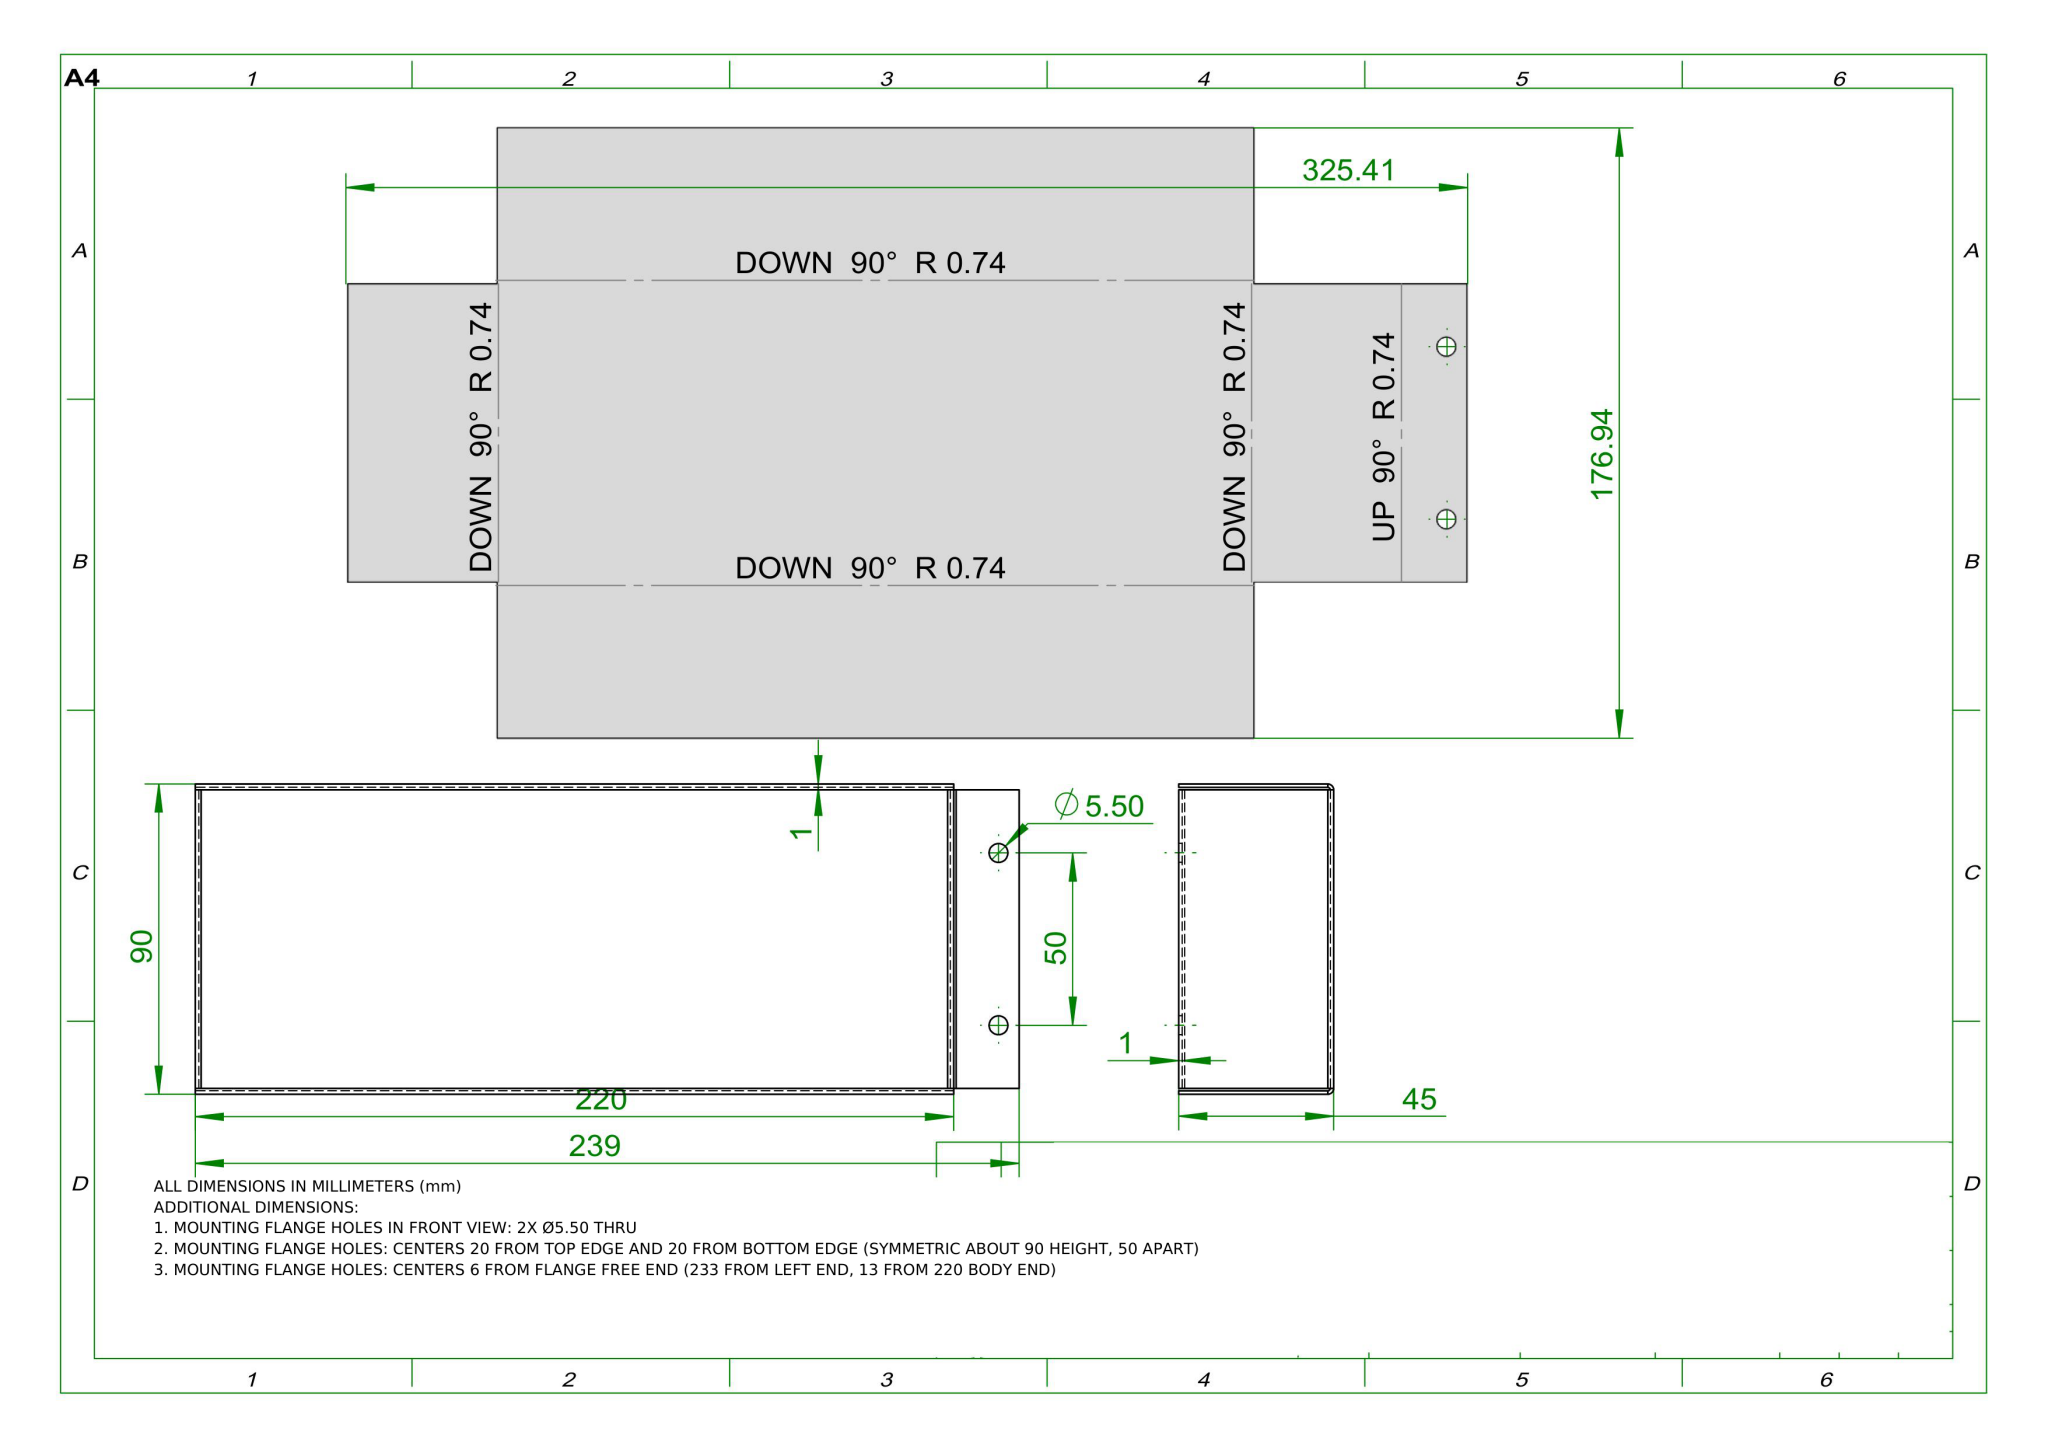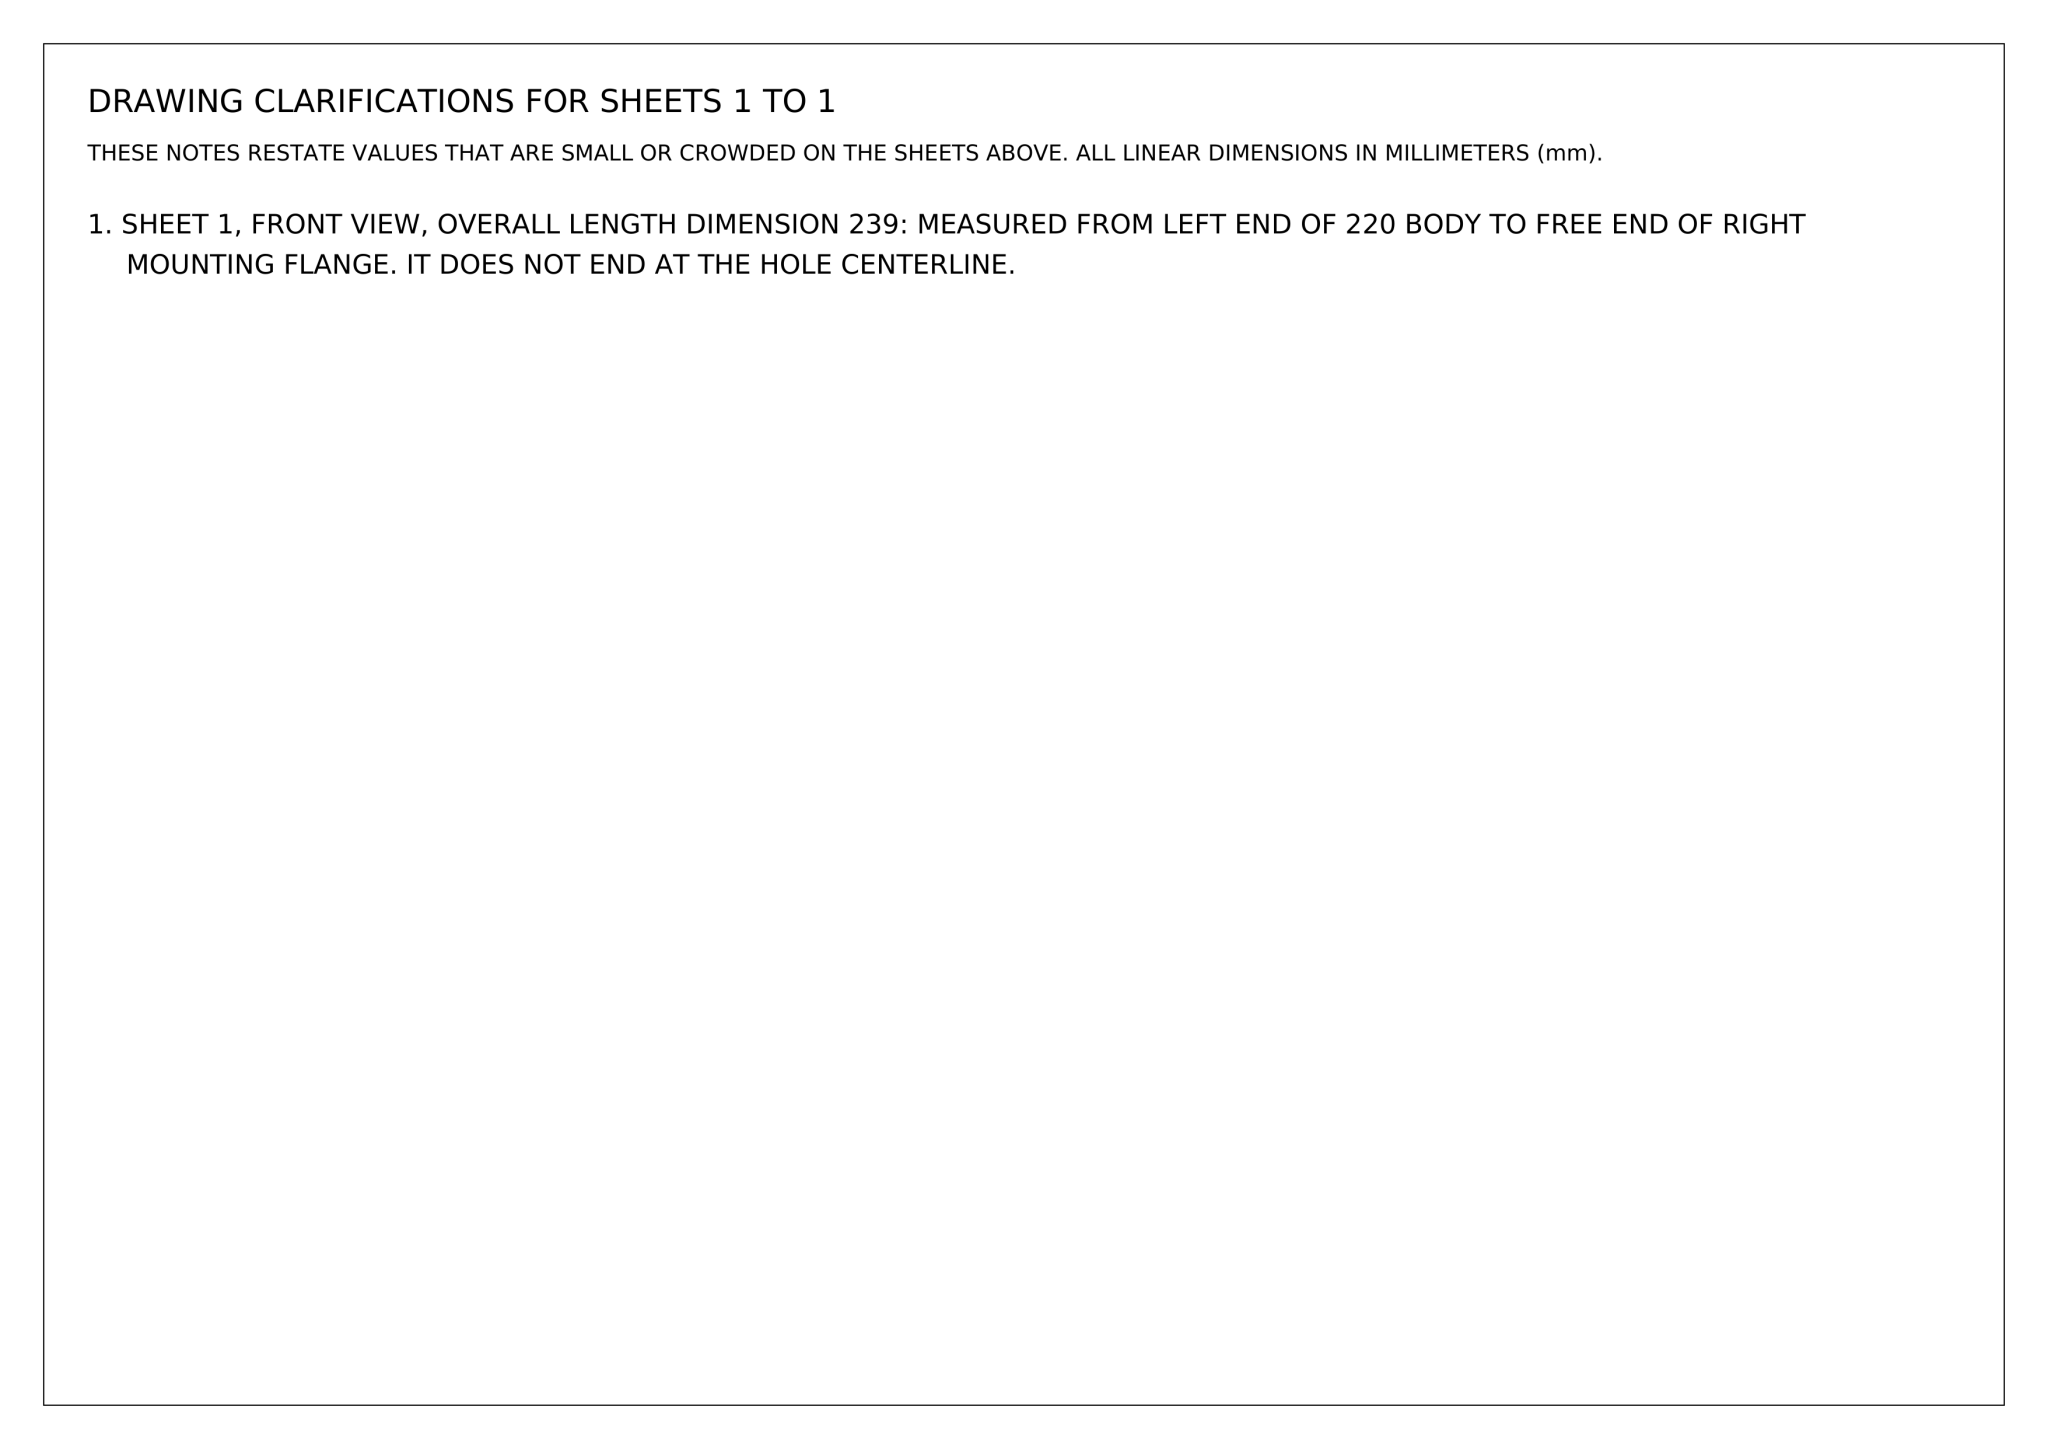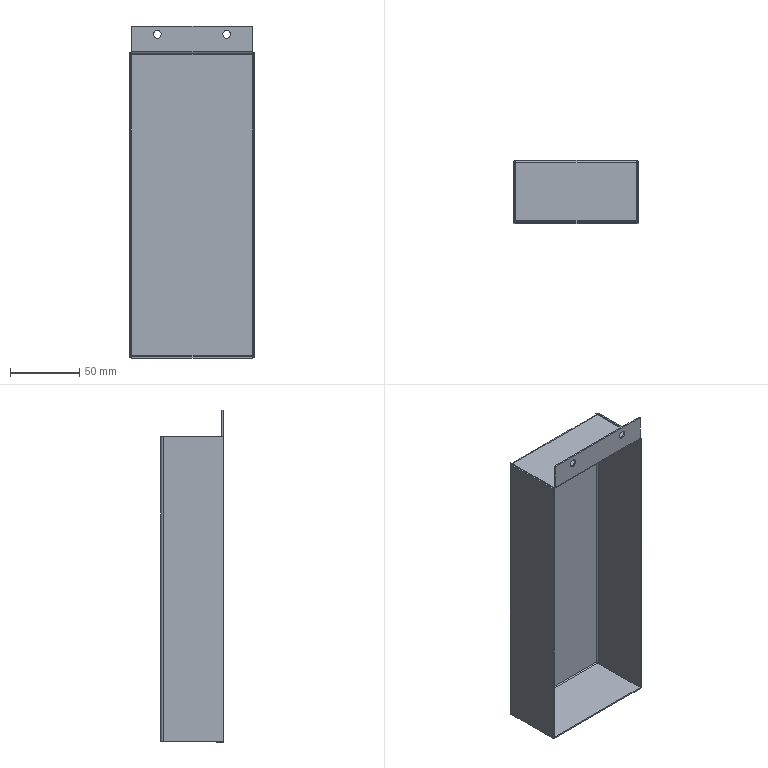Part | NX | mm | 1 solid | 54 faces | box 90 x 45 x 239 mm | volume 48000 mm3 | plane 40 | cylinder 14 | commonest cylinder face diameters 3.473 x5 1.473 x5 5.5 x4